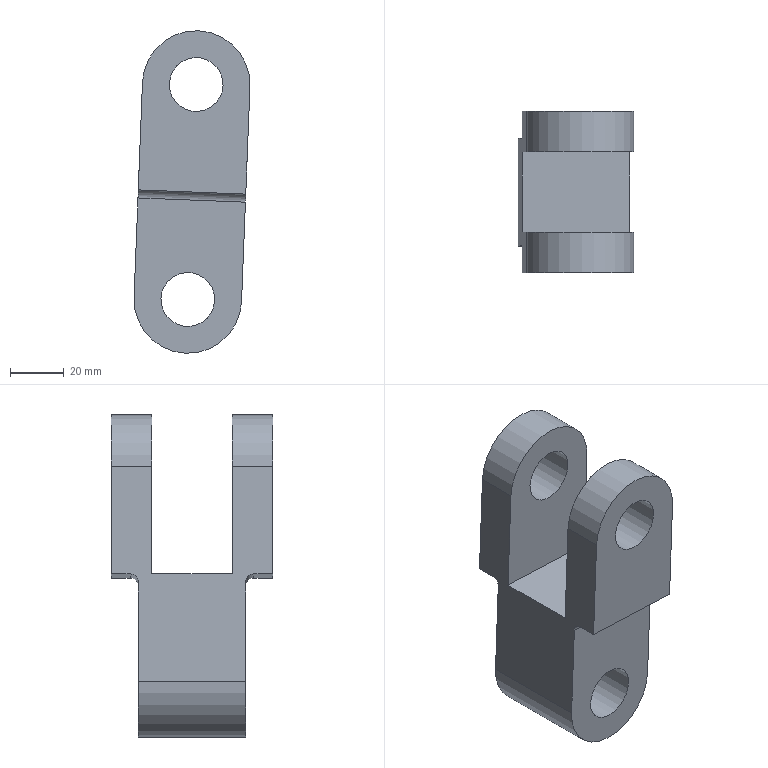Component | NX | SWING_BRACKET | 1 solid | 19 faces | volume 134146 mm3 | plane 11 | cylinder 8 | commonest cylinder face diameters 40 x3 20 x3 6 x2